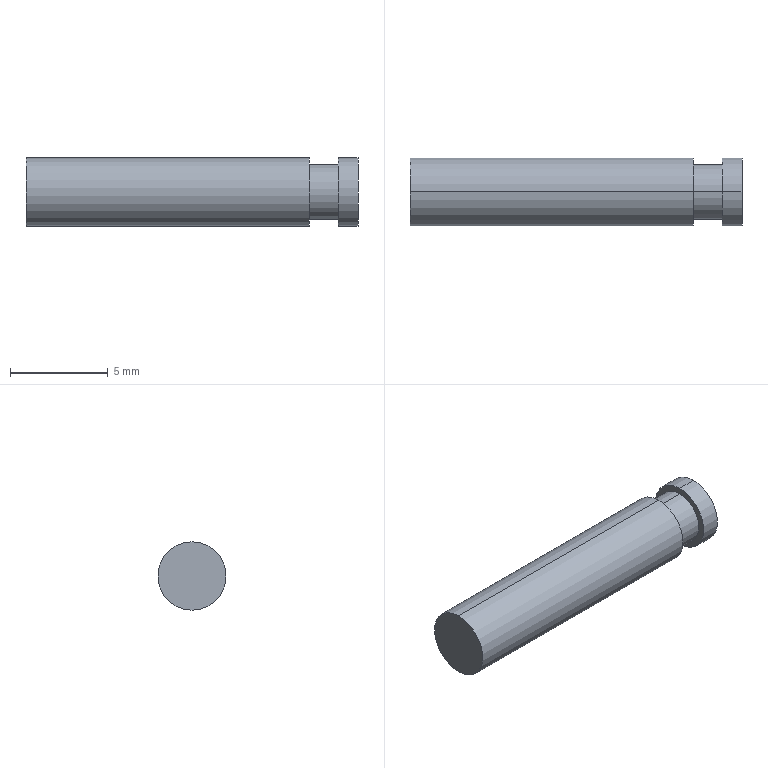Component | SolidWorks | InspectionPart-1 | 1 solid | 10 faces | box 17 x 3.5 x 3.5 mm | volume 158 mm3 | cylinder 6 | plane 4 | commonest cylinder face diameters 3.5 x4 2.8 x2
build123d program:
from build123d import *

# Parameters (mm, degrees)
SKETCH1_R          = 1.75
EXTRUDE1_DEPTH     = 17
CUT_EXTRUDE1_START = -1
SKETCH2_OUTSIDE_W  = 9.042
SKETCH2_OUTSIDE_H  = 9.042
SKETCH2_OUTSIDE_R  = 1.4
CUT_EXTRUDE1_DEPTH = 1.5


with BuildPart() as part:
    # Sketch1 → Extrude1 (new body)
    with BuildSketch(Plane(origin=(0, 0, 0), x_dir=(0, 0, -1), z_dir=(1, 0, 0))):
        Circle(SKETCH1_R)
    extrude(amount=EXTRUDE1_DEPTH)

    # Sketch2 outside → Cut-Extrude1 (cut)
    with BuildSketch(Plane(origin=(17, 0, 0), x_dir=(0, 0, -1), z_dir=(1, 0, 0)).offset(CUT_EXTRUDE1_START)):
        Rectangle(SKETCH2_OUTSIDE_W, SKETCH2_OUTSIDE_H)
        Circle(SKETCH2_OUTSIDE_R, mode=Mode.SUBTRACT)
    extrude(amount=-CUT_EXTRUDE1_DEPTH, mode=Mode.SUBTRACT)


solid = part.part

# Placed as in the assembly
solid = solid.moved(Location((25.117, 79.872, -52.387), (0, 0, 0)))
STEP:
#1=COLOUR_RGB('',0.7922,0.8196,0.9333);
#2=FILL_AREA_STYLE_COLOUR('',#1);
#3=FILL_AREA_STYLE('',(#2));
#4=SURFACE_STYLE_FILL_AREA(#3);
#5=SURFACE_SIDE_STYLE('',(#4));
#6=SURFACE_STYLE_USAGE(.BOTH.,#5);
#7=PRESENTATION_STYLE_ASSIGNMENT((#6));
#8=CARTESIAN_POINT('',(1.658,3.145,-2.131));
#9=VERTEX_POINT('',#8);
#10=CARTESIAN_POINT('',(1.658,3.145,-1.994));
#11=VERTEX_POINT('',#10);
#12=CARTESIAN_POINT('',(1.658,3.145,-2.062));
#13=DIRECTION('',(1.,0.,0.));
#14=DIRECTION('',(0.,0.,-1.));
#15=AXIS2_PLACEMENT_3D('',#12,#13,#14);
#16=CIRCLE('',#15,0.0689);
#17=EDGE_CURVE('',#9,#11,#16,.T.);
#18=ORIENTED_EDGE('',*,*,#17,.F.);
#19=CARTESIAN_POINT('',(1.619,3.145,-2.131));
#20=VERTEX_POINT('',#19);
#21=CARTESIAN_POINT('',(1.658,3.145,-2.131));
#22=DIRECTION('',(-1.,0.,0.));
#23=VECTOR('',#22,39.37);
#24=LINE('',#21,#23);
#25=EDGE_CURVE('',#9,#20,#24,.T.);
#26=ORIENTED_EDGE('',*,*,#25,.T.);
#27=CARTESIAN_POINT('',(1.619,3.145,-1.994));
#28=VERTEX_POINT('',#27);
#29=CARTESIAN_POINT('',(1.619,3.145,-2.062));
#30=DIRECTION('',(1.,0.,0.));
#31=DIRECTION('',(0.,0.,-1.));
#32=AXIS2_PLACEMENT_3D('',#29,#30,#31);
#33=CIRCLE('',#32,0.0689);
#34=EDGE_CURVE('',#20,#28,#33,.T.);
#35=ORIENTED_EDGE('',*,*,#34,.T.);
#36=CARTESIAN_POINT('',(1.658,3.145,-1.994));
#37=DIRECTION('',(-1.,0.,0.));
#38=VECTOR('',#37,39.37);
#39=LINE('',#36,#38);
#40=EDGE_CURVE('',#11,#28,#39,.T.);
#41=ORIENTED_EDGE('',*,*,#40,.F.);
#42=EDGE_LOOP('',(#18,#26,#35,#41));
#43=FACE_OUTER_BOUND('',#42,.T.);
#44=CARTESIAN_POINT('',(1.658,3.145,-2.062));
#45=DIRECTION('',(-1.,0.,0.));
#46=DIRECTION('',(0.,0.,1.));
#47=AXIS2_PLACEMENT_3D('',#44,#45,#46);
#48=CYLINDRICAL_SURFACE('',#47,0.0689);
#49=ADVANCED_FACE('',(#43),#48,.T.);
#50=CARTESIAN_POINT('',(1.56,3.145,-2.118));
#51=VERTEX_POINT('',#50);
#52=CARTESIAN_POINT('',(1.56,3.145,-2.007));
#53=VERTEX_POINT('',#52);
#54=CARTESIAN_POINT('',(1.56,3.145,-2.062));
#55=DIRECTION('',(1.,0.,0.));
#56=DIRECTION('',(0.,0.,-1.));
#57=AXIS2_PLACEMENT_3D('',#54,#55,#56);
#58=CIRCLE('',#57,0.05512);
#59=EDGE_CURVE('',#51,#53,#58,.T.);
#60=ORIENTED_EDGE('',*,*,#59,.T.);
#61=CARTESIAN_POINT('',(1.619,3.145,-2.007));
#62=VERTEX_POINT('',#61);
#63=CARTESIAN_POINT('',(1.56,3.145,-2.007));
#64=DIRECTION('',(1.,0.,0.));
#65=VECTOR('',#64,39.37);
#66=LINE('',#63,#65);
#67=EDGE_CURVE('',#53,#62,#66,.T.);
#68=ORIENTED_EDGE('',*,*,#67,.T.);
#69=CARTESIAN_POINT('',(1.619,3.145,-2.118));
#70=VERTEX_POINT('',#69);
#71=CARTESIAN_POINT('',(1.619,3.145,-2.062));
#72=DIRECTION('',(1.,0.,0.));
#73=DIRECTION('',(0.,0.,-1.));
#74=AXIS2_PLACEMENT_3D('',#71,#72,#73);
#75=CIRCLE('',#74,0.05512);
#76=EDGE_CURVE('',#70,#62,#75,.T.);
#77=ORIENTED_EDGE('',*,*,#76,.F.);
#78=CARTESIAN_POINT('',(1.56,3.145,-2.118));
#79=DIRECTION('',(1.,0.,0.));
#80=VECTOR('',#79,39.37);
#81=LINE('',#78,#80);
#82=EDGE_CURVE('',#51,#70,#81,.T.);
#83=ORIENTED_EDGE('',*,*,#82,.F.);
#84=EDGE_LOOP('',(#60,#68,#77,#83));
#85=FACE_OUTER_BOUND('',#84,.T.);
#86=CARTESIAN_POINT('',(1.56,3.145,-2.062));
#87=DIRECTION('',(1.,0.,0.));
#88=DIRECTION('',(0.,0.,-1.));
#89=AXIS2_PLACEMENT_3D('',#86,#87,#88);
#90=CYLINDRICAL_SURFACE('',#89,0.05512);
#91=ADVANCED_FACE('',(#85),#90,.T.);
#92=CARTESIAN_POINT('',(1.56,3.145,-2.131));
#93=VERTEX_POINT('',#92);
#94=CARTESIAN_POINT('',(1.56,3.145,-1.994));
#95=VERTEX_POINT('',#94);
#96=CARTESIAN_POINT('',(1.56,3.145,-2.062));
#97=DIRECTION('',(1.,0.,0.));
#98=DIRECTION('',(0.,0.,-1.));
#99=AXIS2_PLACEMENT_3D('',#96,#97,#98);
#100=CIRCLE('',#99,0.0689);
#101=EDGE_CURVE('',#93,#95,#100,.T.);
#102=ORIENTED_EDGE('',*,*,#101,.F.);
#103=CARTESIAN_POINT('',(0.9889,3.145,-2.131));
#104=VERTEX_POINT('',#103);
#105=CARTESIAN_POINT('',(1.658,3.145,-2.131));
#106=DIRECTION('',(-1.,0.,0.));
#107=VECTOR('',#106,39.37);
#108=LINE('',#105,#107);
#109=EDGE_CURVE('',#93,#104,#108,.T.);
#110=ORIENTED_EDGE('',*,*,#109,.T.);
#111=CARTESIAN_POINT('',(0.9889,3.145,-1.994));
#112=VERTEX_POINT('',#111);
#113=CARTESIAN_POINT('',(0.9889,3.145,-2.062));
#114=DIRECTION('',(1.,0.,0.));
#115=DIRECTION('',(0.,0.,-1.));
#116=AXIS2_PLACEMENT_3D('',#113,#114,#115);
#117=CIRCLE('',#116,0.0689);
#118=EDGE_CURVE('',#104,#112,#117,.T.);
#119=ORIENTED_EDGE('',*,*,#118,.T.);
#120=CARTESIAN_POINT('',(1.658,3.145,-1.994));
#121=DIRECTION('',(-1.,0.,0.));
#122=VECTOR('',#121,39.37);
#123=LINE('',#120,#122);
#124=EDGE_CURVE('',#95,#112,#123,.T.);
#125=ORIENTED_EDGE('',*,*,#124,.F.);
#126=EDGE_LOOP('',(#102,#110,#119,#125));
#127=FACE_OUTER_BOUND('',#126,.T.);
#128=CARTESIAN_POINT('',(1.658,3.145,-2.062));
#129=DIRECTION('',(-1.,0.,0.));
#130=DIRECTION('',(0.,0.,1.));
#131=AXIS2_PLACEMENT_3D('',#128,#129,#130);
#132=CYLINDRICAL_SURFACE('',#131,0.0689);
#133=ADVANCED_FACE('',(#127),#132,.T.);
#134=ORIENTED_EDGE('',*,*,#109,.F.);
#135=CARTESIAN_POINT('',(1.56,3.145,-2.062));
#136=DIRECTION('',(1.,0.,0.));
#137=DIRECTION('',(0.,0.,-1.));
#138=AXIS2_PLACEMENT_3D('',#135,#136,#137);
#139=CIRCLE('',#138,0.0689);
#140=EDGE_CURVE('',#95,#93,#139,.T.);
#141=ORIENTED_EDGE('',*,*,#140,.F.);
#142=ORIENTED_EDGE('',*,*,#124,.T.);
#143=CARTESIAN_POINT('',(0.9889,3.145,-2.062));
#144=DIRECTION('',(1.,0.,0.));
#145=DIRECTION('',(0.,0.,-1.));
#146=AXIS2_PLACEMENT_3D('',#143,#144,#145);
#147=CIRCLE('',#146,0.0689);
#148=EDGE_CURVE('',#112,#104,#147,.T.);
#149=ORIENTED_EDGE('',*,*,#148,.T.);
#150=EDGE_LOOP('',(#134,#141,#142,#149));
#151=FACE_OUTER_BOUND('',#150,.T.);
#152=CARTESIAN_POINT('',(1.658,3.145,-2.062));
#153=DIRECTION('',(-1.,0.,0.));
#154=DIRECTION('',(0.,0.,1.));
#155=AXIS2_PLACEMENT_3D('',#152,#153,#154);
#156=CYLINDRICAL_SURFACE('',#155,0.0689);
#157=ADVANCED_FACE('',(#151),#156,.T.);
#158=ORIENTED_EDGE('',*,*,#148,.F.);
#159=ORIENTED_EDGE('',*,*,#118,.F.);
#160=EDGE_LOOP('',(#158,#159));
#161=FACE_OUTER_BOUND('',#160,.T.);
#162=CARTESIAN_POINT('',(0.9889,3.145,-2.062));
#163=DIRECTION('',(1.,0.,0.));
#164=DIRECTION('',(0.,0.,-1.));
#165=AXIS2_PLACEMENT_3D('',#162,#163,#164);
#166=PLANE('',#165);
#167=ADVANCED_FACE('',(#161),#166,.F.);
#168=ORIENTED_EDGE('',*,*,#59,.F.);
#169=CARTESIAN_POINT('',(1.56,3.145,-2.062));
#170=DIRECTION('',(1.,0.,0.));
#171=DIRECTION('',(0.,0.,-1.));
#172=AXIS2_PLACEMENT_3D('',#169,#170,#171);
#173=CIRCLE('',#172,0.05512);
#174=EDGE_CURVE('',#53,#51,#173,.T.);
#175=ORIENTED_EDGE('',*,*,#174,.F.);
#176=EDGE_LOOP('',(#168,#175));
#177=FACE_BOUND('',#176,.T.);
#178=ORIENTED_EDGE('',*,*,#140,.T.);
#179=ORIENTED_EDGE('',*,*,#101,.T.);
#180=EDGE_LOOP('',(#178,#179));
#181=FACE_OUTER_BOUND('',#180,.T.);
#182=CARTESIAN_POINT('',(1.56,3.145,-2.062));
#183=DIRECTION('',(1.,0.,0.));
#184=DIRECTION('',(0.,0.,-1.));
#185=AXIS2_PLACEMENT_3D('',#182,#183,#184);
#186=PLANE('',#185);
#187=ADVANCED_FACE('',(#177,#181),#186,.T.);
#188=ORIENTED_EDGE('',*,*,#76,.T.);
#189=CARTESIAN_POINT('',(1.619,3.145,-2.062));
#190=DIRECTION('',(1.,0.,0.));
#191=DIRECTION('',(0.,0.,-1.));
#192=AXIS2_PLACEMENT_3D('',#189,#190,#191);
#193=CIRCLE('',#192,0.05512);
#194=EDGE_CURVE('',#62,#70,#193,.T.);
#195=ORIENTED_EDGE('',*,*,#194,.T.);
#196=EDGE_LOOP('',(#188,#195));
#197=FACE_BOUND('',#196,.T.);
#198=CARTESIAN_POINT('',(1.619,3.145,-2.062));
#199=DIRECTION('',(1.,0.,0.));
#200=DIRECTION('',(0.,0.,-1.));
#201=AXIS2_PLACEMENT_3D('',#198,#199,#200);
#202=CIRCLE('',#201,0.0689);
#203=EDGE_CURVE('',#28,#20,#202,.T.);
#204=ORIENTED_EDGE('',*,*,#203,.F.);
#205=ORIENTED_EDGE('',*,*,#34,.F.);
#206=EDGE_LOOP('',(#204,#205));
#207=FACE_OUTER_BOUND('',#206,.T.);
#208=CARTESIAN_POINT('',(1.619,3.145,-2.062));
#209=DIRECTION('',(1.,0.,0.));
#210=DIRECTION('',(0.,0.,-1.));
#211=AXIS2_PLACEMENT_3D('',#208,#209,#210);
#212=PLANE('',#211);
#213=ADVANCED_FACE('',(#197,#207),#212,.F.);
#214=ORIENTED_EDGE('',*,*,#67,.F.);
#215=ORIENTED_EDGE('',*,*,#174,.T.);
#216=ORIENTED_EDGE('',*,*,#82,.T.);
#217=ORIENTED_EDGE('',*,*,#194,.F.);
#218=EDGE_LOOP('',(#214,#215,#216,#217));
#219=FACE_OUTER_BOUND('',#218,.T.);
#220=CARTESIAN_POINT('',(1.56,3.145,-2.062));
#221=DIRECTION('',(1.,0.,0.));
#222=DIRECTION('',(0.,0.,-1.));
#223=AXIS2_PLACEMENT_3D('',#220,#221,#222);
#224=CYLINDRICAL_SURFACE('',#223,0.05512);
#225=ADVANCED_FACE('',(#219),#224,.T.);
#226=CARTESIAN_POINT('',(1.658,3.145,-2.062));
#227=DIRECTION('',(1.,0.,0.));
#228=DIRECTION('',(0.,0.,-1.));
#229=AXIS2_PLACEMENT_3D('',#226,#227,#228);
#230=CIRCLE('',#229,0.0689);
#231=EDGE_CURVE('',#11,#9,#230,.T.);
#232=ORIENTED_EDGE('',*,*,#231,.T.);
#233=ORIENTED_EDGE('',*,*,#17,.T.);
#234=EDGE_LOOP('',(#232,#233));
#235=FACE_OUTER_BOUND('',#234,.T.);
#236=CARTESIAN_POINT('',(1.658,3.145,-2.062));
#237=DIRECTION('',(1.,0.,0.));
#238=DIRECTION('',(0.,0.,-1.));
#239=AXIS2_PLACEMENT_3D('',#236,#237,#238);
#240=PLANE('',#239);
#241=ADVANCED_FACE('',(#235),#240,.T.);
#242=ORIENTED_EDGE('',*,*,#25,.F.);
#243=ORIENTED_EDGE('',*,*,#231,.F.);
#244=ORIENTED_EDGE('',*,*,#40,.T.);
#245=ORIENTED_EDGE('',*,*,#203,.T.);
#246=EDGE_LOOP('',(#242,#243,#244,#245));
#247=FACE_OUTER_BOUND('',#246,.T.);
#248=CARTESIAN_POINT('',(1.658,3.145,-2.062));
#249=DIRECTION('',(-1.,0.,0.));
#250=DIRECTION('',(0.,0.,1.));
#251=AXIS2_PLACEMENT_3D('',#248,#249,#250);
#252=CYLINDRICAL_SURFACE('',#251,0.0689);
#253=ADVANCED_FACE('',(#247),#252,.T.);
#254=CLOSED_SHELL('',(#49,#91,#133,#157,#167,#187,#213,#225,#241,#253));
#255=MANIFOLD_SOLID_BREP('',#254);
#256=STYLED_ITEM('',(#7),#255);
#257=PRESENTATION_LAYER_ASSIGNMENT('','',(#256));
#258=(LENGTH_UNIT()NAMED_UNIT(*)SI_UNIT($,.METRE.));
#259=LENGTH_MEASURE_WITH_UNIT(LENGTH_MEASURE(0.0254),#258);
#260=DIMENSIONAL_EXPONENTS(1.,0.,0.,0.,0.,0.,0.);
#261=(CONVERSION_BASED_UNIT('',#259)LENGTH_UNIT()NAMED_UNIT(#260));
#262=UNCERTAINTY_MEASURE_WITH_UNIT(LENGTH_MEASURE(0.00001),#261,'','');
#263=(NAMED_UNIT(*)PLANE_ANGLE_UNIT()SI_UNIT($,.RADIAN.));
#264=(NAMED_UNIT(*)SI_UNIT($,.STERADIAN.)SOLID_ANGLE_UNIT());
#265=(GEOMETRIC_REPRESENTATION_CONTEXT(3)GLOBAL_UNCERTAINTY_ASSIGNED_CONTEXT((#262))GLOBAL_UNIT_ASSIGNED_CONTEXT((#261,#263,#264))REPRESENTATION_CONTEXT('',''));
#266=MECHANICAL_DESIGN_GEOMETRIC_PRESENTATION_REPRESENTATION('',(#256),#265);
#267=CARTESIAN_POINT('',(0.,0.,0.));
#268=DIRECTION('',(0.,0.,1.));
#269=DIRECTION('',(1.,0.,0.));
#270=AXIS2_PLACEMENT_3D('',#267,#268,#269);
#271=(LENGTH_UNIT()NAMED_UNIT(*)SI_UNIT($,.METRE.));
#272=LENGTH_MEASURE_WITH_UNIT(LENGTH_MEASURE(0.0254),#271);
#273=DIMENSIONAL_EXPONENTS(1.,0.,0.,0.,0.,0.,0.);
#274=(CONVERSION_BASED_UNIT('',#272)LENGTH_UNIT()NAMED_UNIT(#273));
#275=UNCERTAINTY_MEASURE_WITH_UNIT(LENGTH_MEASURE(0.00001),#274,'','');
#276=(NAMED_UNIT(*)PLANE_ANGLE_UNIT()SI_UNIT($,.RADIAN.));
#277=(NAMED_UNIT(*)SI_UNIT($,.STERADIAN.)SOLID_ANGLE_UNIT());
#278=(GEOMETRIC_REPRESENTATION_CONTEXT(3)GLOBAL_UNCERTAINTY_ASSIGNED_CONTEXT((#275))GLOBAL_UNIT_ASSIGNED_CONTEXT((#274,#276,#277))REPRESENTATION_CONTEXT('',''));
#279=ADVANCED_BREP_SHAPE_REPRESENTATION('',(#255,#270),#278);